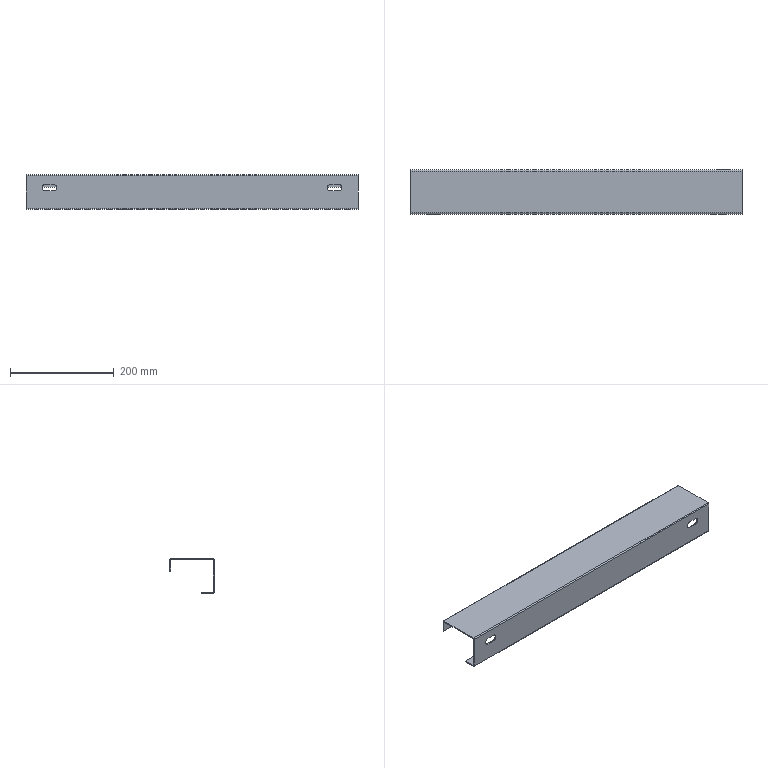Component | SolidWorks | KSHE-016.004-1 | 1 solid | 104 faces | volume 240855 mm3 | cylinder 74 | plane 30 | commonest cylinder face diameters 9 x64 13 x4 4.2 x3 0.2 x3